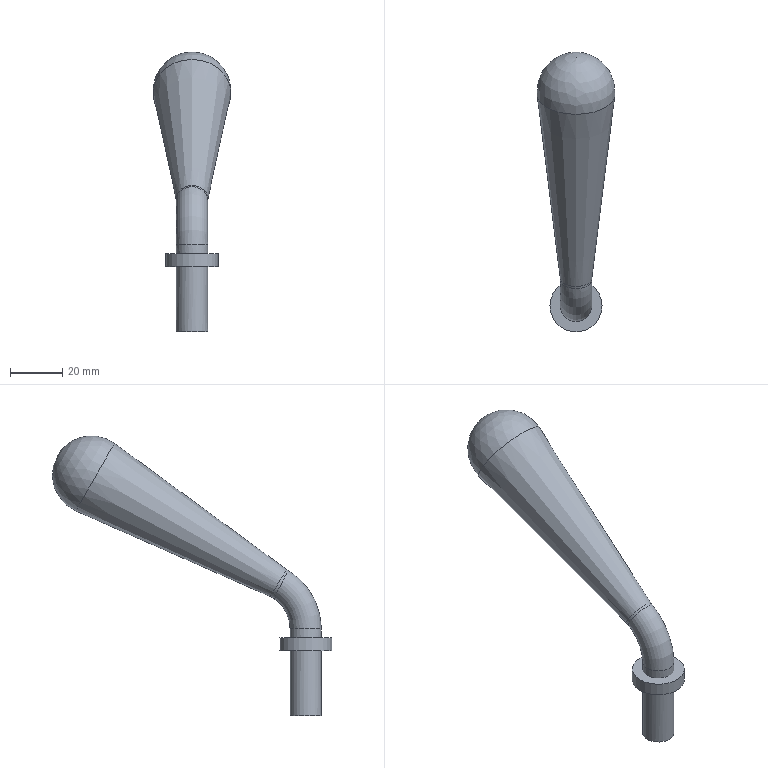Component | NX | LOCK_HANDLE | 1 solid | 10 faces | box 30 x 107.27 x 107.5 mm | volume 45177 mm3 | cylinder 3 | plane 3 | torus 1 | sphere 1 | cone 1 | spline 1 | commonest cylinder face diameters 12 x2 20 x1
STEP:
#1=CARTESIAN_POINT('',(0.,0.,0.));
#2=DIRECTION('',(0.,0.,1.));
#3=DIRECTION('',(1.,0.,0.));
#4=AXIS2_PLACEMENT_3D('',#1,#2,#3);
#5=CARTESIAN_POINT('',(36.,50.,164.5));
#6=VERTEX_POINT('',#5);
#7=CARTESIAN_POINT('',(42.,44.,164.5));
#8=VERTEX_POINT('',#7);
#9=CARTESIAN_POINT('',(36.,44.,164.5));
#10=DIRECTION('',(0.,0.,-1.));
#11=DIRECTION('',(1.,0.,0.));
#12=AXIS2_PLACEMENT_3D('',#9,#10,#11);
#13=CIRCLE('',#12,6.);
#14=CARTESIAN_POINT('',(36.,44.,167.953));
#15=DIRECTION('',(0.,0.,-1.));
#16=DIRECTION('',(-1.,0.,0.));
#17=AXIS2_PLACEMENT_3D('',#14,#15,#16);
#18=CYLINDRICAL_SURFACE('',#17,6.);
#19=CARTESIAN_POINT('',(-3.142,3.453));
#20=DIRECTION('',(1.,0.));
#21=VECTOR('',#20,1.);
#22=LINE('',#19,#21);
#23=(GEOMETRIC_REPRESENTATION_CONTEXT(2)PARAMETRIC_REPRESENTATION_CONTEXT()REPRESENTATION_CONTEXT('',''));
#24=DEFINITIONAL_REPRESENTATION('',(#22),#23);
#25=PCURVE('',#18,#24);
#26=CARTESIAN_POINT('',(36.,44.,164.5));
#27=DIRECTION('',(0.,0.,1.));
#28=DIRECTION('',(1.,0.,0.));
#29=AXIS2_PLACEMENT_3D('',#26,#27,#28);
#30=PLANE('',#29);
#31=CARTESIAN_POINT('',(6.,0.));
#32=CARTESIAN_POINT('',(6.,-10.392));
#33=CARTESIAN_POINT('',(-3.,-5.196));
#34=CARTESIAN_POINT('',(-12.,-0.));
#35=CARTESIAN_POINT('',(-3.,5.196));
#36=CARTESIAN_POINT('',(6.,10.392));
#37=CARTESIAN_POINT('',(6.,0.));
#38=(BOUNDED_CURVE()B_SPLINE_CURVE(2,(#31,#32,#33,#34,#35,#36,#37),.UNSPECIFIED.,.T.,.F.)B_SPLINE_CURVE_WITH_KNOTS((1,2,2,2,2,1),(-2.094,0.,2.094,4.189,6.283,8.378),.UNSPECIFIED.)CURVE()GEOMETRIC_REPRESENTATION_ITEM()RATIONAL_B_SPLINE_CURVE((1.,0.5,1.,0.5,1.,0.5,1.))REPRESENTATION_ITEM(''));
#39=(GEOMETRIC_REPRESENTATION_CONTEXT(2)PARAMETRIC_REPRESENTATION_CONTEXT()REPRESENTATION_CONTEXT('',''));
#40=DEFINITIONAL_REPRESENTATION('',(#38),#39);
#41=PCURVE('',#30,#40);
#42=SURFACE_CURVE('',#13,(#25,#41),.PCURVE_S1.);
#43=EDGE_CURVE('',#6,#8,#42,.T.);
#44=ORIENTED_EDGE('',*,*,#43,.F.);
#45=CARTESIAN_POINT('',(36.,50.,167.953));
#46=VERTEX_POINT('',#45);
#47=CARTESIAN_POINT('',(36.,50.,167.953));
#48=CARTESIAN_POINT('',(36.,50.,164.5));
#49=B_SPLINE_CURVE_WITH_KNOTS('',1,(#47,#48),.UNSPECIFIED.,.F.,.F.,(2,2),(0.,3.453),.PIECEWISE_BEZIER_KNOTS.);
#50=CARTESIAN_POINT('',(1.571,0.));
#51=DIRECTION('',(0.,1.));
#52=VECTOR('',#51,1.);
#53=LINE('',#50,#52);
#54=(GEOMETRIC_REPRESENTATION_CONTEXT(2)PARAMETRIC_REPRESENTATION_CONTEXT()REPRESENTATION_CONTEXT('',''));
#55=DEFINITIONAL_REPRESENTATION('',(#53),#54);
#56=PCURVE('',#18,#55);
#57=CARTESIAN_POINT('',(7.854,0.));
#58=DIRECTION('',(0.,1.));
#59=VECTOR('',#58,1.);
#60=LINE('',#57,#59);
#61=(GEOMETRIC_REPRESENTATION_CONTEXT(2)PARAMETRIC_REPRESENTATION_CONTEXT()REPRESENTATION_CONTEXT('',''));
#62=DEFINITIONAL_REPRESENTATION('',(#60),#61);
#63=PCURVE('',#18,#62);
#64=SEAM_CURVE('',#49,(#56,#63),.PCURVE_S1.);
#65=EDGE_CURVE('',#46,#6,#64,.T.);
#66=ORIENTED_EDGE('',*,*,#65,.F.);
#67=CARTESIAN_POINT('',(36.,38.,167.953));
#68=VERTEX_POINT('',#67);
#69=CARTESIAN_POINT('',(36.,44.,167.953));
#70=DIRECTION('',(0.,-0.,-1.));
#71=DIRECTION('',(0.,1.,-0.));
#72=AXIS2_PLACEMENT_3D('',#69,#70,#71);
#73=CIRCLE('',#72,6.);
#74=CARTESIAN_POINT('',(1.571,0.));
#75=DIRECTION('',(1.,0.));
#76=VECTOR('',#75,1.);
#77=LINE('',#74,#76);
#78=(GEOMETRIC_REPRESENTATION_CONTEXT(2)PARAMETRIC_REPRESENTATION_CONTEXT()REPRESENTATION_CONTEXT('',''));
#79=DEFINITIONAL_REPRESENTATION('',(#77),#78);
#80=PCURVE('',#18,#79);
#81=CARTESIAN_POINT('',(36.,64.,167.953));
#82=DIRECTION('',(-1.,0.,0.));
#83=DIRECTION('',(0.,0.,1.));
#84=AXIS2_PLACEMENT_3D('',#81,#82,#83);
#85=TOROIDAL_SURFACE('',#84,20.,6.);
#86=CARTESIAN_POINT('',(4.712,3.142));
#87=DIRECTION('',(0.,1.));
#88=VECTOR('',#87,1.);
#89=LINE('',#86,#88);
#90=(GEOMETRIC_REPRESENTATION_CONTEXT(2)PARAMETRIC_REPRESENTATION_CONTEXT()REPRESENTATION_CONTEXT('',''));
#91=DEFINITIONAL_REPRESENTATION('',(#89),#90);
#92=PCURVE('',#85,#91);
#93=SURFACE_CURVE('',#73,(#80,#92),.PCURVE_S1.);
#94=EDGE_CURVE('',#46,#68,#93,.T.);
#95=ORIENTED_EDGE('',*,*,#94,.T.);
#96=CARTESIAN_POINT('',(36.,44.,167.953));
#97=DIRECTION('',(0.,-0.,-1.));
#98=DIRECTION('',(0.,1.,-0.));
#99=AXIS2_PLACEMENT_3D('',#96,#97,#98);
#100=CIRCLE('',#99,6.);
#101=CARTESIAN_POINT('',(1.571,0.));
#102=DIRECTION('',(1.,0.));
#103=VECTOR('',#102,1.);
#104=LINE('',#101,#103);
#105=(GEOMETRIC_REPRESENTATION_CONTEXT(2)PARAMETRIC_REPRESENTATION_CONTEXT()REPRESENTATION_CONTEXT('',''));
#106=DEFINITIONAL_REPRESENTATION('',(#104),#105);
#107=PCURVE('',#18,#106);
#108=CARTESIAN_POINT('',(4.712,-3.142));
#109=DIRECTION('',(0.,1.));
#110=VECTOR('',#109,1.);
#111=LINE('',#108,#110);
#112=(GEOMETRIC_REPRESENTATION_CONTEXT(2)PARAMETRIC_REPRESENTATION_CONTEXT()REPRESENTATION_CONTEXT('',''));
#113=DEFINITIONAL_REPRESENTATION('',(#111),#112);
#114=PCURVE('',#85,#113);
#115=SURFACE_CURVE('',#100,(#107,#114),.PCURVE_S1.);
#116=EDGE_CURVE('',#68,#46,#115,.T.);
#117=ORIENTED_EDGE('',*,*,#116,.T.);
#118=ORIENTED_EDGE('',*,*,#65,.T.);
#119=CARTESIAN_POINT('',(36.,44.,164.5));
#120=DIRECTION('',(0.,0.,-1.));
#121=DIRECTION('',(1.,0.,0.));
#122=AXIS2_PLACEMENT_3D('',#119,#120,#121);
#123=CIRCLE('',#122,6.);
#124=CARTESIAN_POINT('',(3.142,3.453));
#125=DIRECTION('',(1.,0.));
#126=VECTOR('',#125,1.);
#127=LINE('',#124,#126);
#128=(GEOMETRIC_REPRESENTATION_CONTEXT(2)PARAMETRIC_REPRESENTATION_CONTEXT()REPRESENTATION_CONTEXT('',''));
#129=DEFINITIONAL_REPRESENTATION('',(#127),#128);
#130=PCURVE('',#18,#129);
#131=CARTESIAN_POINT('',(6.,0.));
#132=CARTESIAN_POINT('',(6.,-10.392));
#133=CARTESIAN_POINT('',(-3.,-5.196));
#134=CARTESIAN_POINT('',(-12.,-0.));
#135=CARTESIAN_POINT('',(-3.,5.196));
#136=CARTESIAN_POINT('',(6.,10.392));
#137=CARTESIAN_POINT('',(6.,0.));
#138=(BOUNDED_CURVE()B_SPLINE_CURVE(2,(#131,#132,#133,#134,#135,#136,#137),.UNSPECIFIED.,.T.,.F.)B_SPLINE_CURVE_WITH_KNOTS((1,2,2,2,2,1),(-2.094,0.,2.094,4.189,6.283,8.378),.UNSPECIFIED.)CURVE()GEOMETRIC_REPRESENTATION_ITEM()RATIONAL_B_SPLINE_CURVE((1.,0.5,1.,0.5,1.,0.5,1.))REPRESENTATION_ITEM(''));
#139=(GEOMETRIC_REPRESENTATION_CONTEXT(2)PARAMETRIC_REPRESENTATION_CONTEXT()REPRESENTATION_CONTEXT('',''));
#140=DEFINITIONAL_REPRESENTATION('',(#138),#139);
#141=PCURVE('',#30,#140);
#142=SURFACE_CURVE('',#123,(#130,#141),.PCURVE_S1.);
#143=EDGE_CURVE('',#8,#6,#142,.T.);
#144=ORIENTED_EDGE('',*,*,#143,.F.);
#145=EDGE_LOOP('',(#44,#66,#95,#117,#118,#144));
#146=FACE_BOUND('',#145,.T.);
#147=ADVANCED_FACE('',(#146),#18,.T.);
#148=CARTESIAN_POINT('',(36.,50.635,190.255));
#149=VERTEX_POINT('',#148);
#150=CARTESIAN_POINT('',(37.592,50.635,190.255));
#151=CARTESIAN_POINT('',(34.408,50.635,190.255));
#152=CARTESIAN_POINT('',(32.847,50.958,189.681));
#153=CARTESIAN_POINT('',(30.634,52.045,187.731));
#154=CARTESIAN_POINT('',(29.99,52.804,186.366));
#155=CARTESIAN_POINT('',(30.01,54.3,183.557));
#156=CARTESIAN_POINT('',(30.675,55.003,182.174));
#157=CARTESIAN_POINT('',(32.89,55.827,180.099));
#158=CARTESIAN_POINT('',(34.423,55.885,179.356));
#159=CARTESIAN_POINT('',(37.609,55.884,179.366));
#160=CARTESIAN_POINT('',(39.13,55.824,180.111));
#161=CARTESIAN_POINT('',(41.334,54.995,182.189));
#162=CARTESIAN_POINT('',(41.993,54.285,183.586));
#163=CARTESIAN_POINT('',(42.007,52.809,186.356));
#164=CARTESIAN_POINT('',(41.375,52.049,187.725));
#165=CARTESIAN_POINT('',(39.136,50.951,189.693));
#166=CARTESIAN_POINT('',(37.592,50.635,190.255));
#167=CARTESIAN_POINT('',(34.408,50.635,190.255));
#168=B_SPLINE_CURVE_WITH_KNOTS('',3,(#150,#151,#152,#153,#154,#155,#156,#157,#158,#159,#160,#161,#162,#163,#164,#165,#166,#167),.UNSPECIFIED.,.T.,.F.,(2,2,2,2,2,2,2,2,2,2,2),(-0.125,0.,0.125,0.25,0.375,0.5,0.625,0.75,0.875,1.,1.125),.UNSPECIFIED.);
#169=CARTESIAN_POINT('',(5.743,0.));
#170=CARTESIAN_POINT('',(5.743,0.04821));
#171=CARTESIAN_POINT('',(5.743,0.1444));
#172=CARTESIAN_POINT('',(5.743,0.2882));
#173=CARTESIAN_POINT('',(5.743,0.4318));
#174=CARTESIAN_POINT('',(5.742,0.575));
#175=CARTESIAN_POINT('',(5.742,0.7179));
#176=CARTESIAN_POINT('',(5.741,0.8607));
#177=CARTESIAN_POINT('',(5.74,1.003));
#178=CARTESIAN_POINT('',(5.738,1.146));
#179=CARTESIAN_POINT('',(5.737,1.29));
#180=CARTESIAN_POINT('',(5.735,1.433));
#181=CARTESIAN_POINT('',(5.732,1.577));
#182=CARTESIAN_POINT('',(5.729,1.721));
#183=CARTESIAN_POINT('',(5.726,1.864));
#184=CARTESIAN_POINT('',(5.722,2.007));
#185=CARTESIAN_POINT('',(5.716,2.15));
#186=CARTESIAN_POINT('',(5.71,2.291));
#187=CARTESIAN_POINT('',(5.702,2.433));
#188=CARTESIAN_POINT('',(5.693,2.574));
#189=CARTESIAN_POINT('',(5.683,2.716));
#190=CARTESIAN_POINT('',(5.673,2.858));
#191=CARTESIAN_POINT('',(5.667,3.));
#192=CARTESIAN_POINT('',(5.664,3.144));
#193=CARTESIAN_POINT('',(5.667,3.288));
#194=CARTESIAN_POINT('',(5.674,3.43));
#195=CARTESIAN_POINT('',(5.683,3.572));
#196=CARTESIAN_POINT('',(5.693,3.713));
#197=CARTESIAN_POINT('',(5.702,3.854));
#198=CARTESIAN_POINT('',(5.71,3.995));
#199=CARTESIAN_POINT('',(5.716,4.137));
#200=CARTESIAN_POINT('',(5.722,4.28));
#201=CARTESIAN_POINT('',(5.726,4.423));
#202=CARTESIAN_POINT('',(5.73,4.565));
#203=CARTESIAN_POINT('',(5.732,4.708));
#204=CARTESIAN_POINT('',(5.735,4.85));
#205=CARTESIAN_POINT('',(5.737,4.993));
#206=CARTESIAN_POINT('',(5.738,5.136));
#207=CARTESIAN_POINT('',(5.74,5.279));
#208=CARTESIAN_POINT('',(5.741,5.423));
#209=CARTESIAN_POINT('',(5.742,5.567));
#210=CARTESIAN_POINT('',(5.742,5.71));
#211=CARTESIAN_POINT('',(5.743,5.853));
#212=CARTESIAN_POINT('',(5.743,5.996));
#213=CARTESIAN_POINT('',(5.743,6.139));
#214=CARTESIAN_POINT('',(5.743,6.235));
#215=CARTESIAN_POINT('',(5.743,6.283));
#216=B_SPLINE_CURVE_WITH_KNOTS('',3,(#169,#170,#171,#172,#173,#174,#175,#176,#177,#178,#179,#180,#181,#182,#183,#184,#185,#186,#187,#188,#189,#190,#191,#192,#193,#194,#195,#196,#197,#198,#199,#200,#201,#202,#203,#204,#205,#206,#207,#208,#209,#210,#211,#212,#213,#214,#215),.UNSPECIFIED.,.F.,.F.,(4,1,1,1,1,1,1,1,1,1,1,1,1,1,1,1,1,1,1,1,1,1,1,1,1,1,1,1,1,1,1,1,1,1,1,1,1,1,1,1,1,1,1,1,4),(0.,0.02273,0.04545,0.06818,0.09091,0.1136,0.1364,0.1591,0.1818,0.2045,0.2273,0.25,0.2727,0.2955,0.3182,0.3409,0.3636,0.3864,0.4091,0.4318,0.4545,0.4773,0.5,0.5227,0.5455,0.5682,0.5909,0.6136,0.6364,0.6591,0.6818,0.7045,0.7273,0.75,0.7727,0.7955,0.8182,0.8409,0.8636,0.8864,0.9091,0.9318,0.9545,0.9773,1.),.QUASI_UNIFORM_KNOTS.);
#217=(GEOMETRIC_REPRESENTATION_CONTEXT(2)PARAMETRIC_REPRESENTATION_CONTEXT()REPRESENTATION_CONTEXT('',''));
#218=DEFINITIONAL_REPRESENTATION('',(#216),#217);
#219=PCURVE('',#85,#218);
#220=CARTESIAN_POINT('',(36.634,50.651,190.225));
#221=CARTESIAN_POINT('',(36.635,51.047,190.463));
#222=CARTESIAN_POINT('',(36.64,51.42,190.735));
#223=CARTESIAN_POINT('',(37.423,50.692,190.152));
#224=CARTESIAN_POINT('',(37.425,51.089,190.39));
#225=CARTESIAN_POINT('',(37.436,51.462,190.662));
#226=CARTESIAN_POINT('',(38.18,50.809,189.945));
#227=CARTESIAN_POINT('',(38.183,51.207,190.183));
#228=CARTESIAN_POINT('',(38.2,51.583,190.455));
#229=CARTESIAN_POINT('',(39.216,51.085,189.452));
#230=CARTESIAN_POINT('',(39.22,51.488,189.692));
#231=CARTESIAN_POINT('',(39.246,51.87,189.963));
#232=CARTESIAN_POINT('',(39.54,51.192,189.26));
#233=CARTESIAN_POINT('',(39.543,51.597,189.501));
#234=CARTESIAN_POINT('',(39.573,51.982,189.771));
#235=CARTESIAN_POINT('',(40.142,51.437,188.822));
#236=CARTESIAN_POINT('',(40.146,51.847,189.064));
#237=CARTESIAN_POINT('',(40.181,52.238,189.334));
#238=CARTESIAN_POINT('',(40.422,51.576,188.573));
#239=CARTESIAN_POINT('',(40.426,51.989,188.817));
#240=CARTESIAN_POINT('',(40.464,52.383,189.086));
#241=CARTESIAN_POINT('',(41.16,52.02,187.774));
#242=CARTESIAN_POINT('',(41.164,52.442,188.022));
#243=CARTESIAN_POINT('',(41.209,52.849,188.29));
#244=CARTESIAN_POINT('',(41.534,52.366,187.15));
#245=CARTESIAN_POINT('',(41.537,52.796,187.401));
#246=CARTESIAN_POINT('',(41.587,53.213,187.669));
#247=CARTESIAN_POINT('',(41.976,53.085,185.833));
#248=CARTESIAN_POINT('',(41.978,53.537,186.096));
#249=CARTESIAN_POINT('',(42.034,53.981,186.365));
#250=CARTESIAN_POINT('',(42.049,53.467,185.126));
#251=CARTESIAN_POINT('',(42.05,53.932,185.397));
#252=CARTESIAN_POINT('',(42.108,54.393,185.668));
#253=CARTESIAN_POINT('',(41.884,54.193,183.746));
#254=CARTESIAN_POINT('',(41.881,54.692,184.038));
#255=CARTESIAN_POINT('',(41.943,55.196,184.316));
#256=CARTESIAN_POINT('',(41.647,54.542,183.061));
#257=CARTESIAN_POINT('',(41.641,55.063,183.368));
#258=CARTESIAN_POINT('',(41.704,55.594,183.652));
#259=CARTESIAN_POINT('',(40.896,55.14,181.806));
#260=CARTESIAN_POINT('',(40.884,55.717,182.155));
#261=CARTESIAN_POINT('',(40.947,56.317,182.457));
#262=CARTESIAN_POINT('',(40.388,55.387,181.238));
#263=CARTESIAN_POINT('',(40.373,55.998,181.615));
#264=CARTESIAN_POINT('',(40.435,56.642,181.93));
#265=CARTESIAN_POINT('',(39.157,55.732,180.273));
#266=CARTESIAN_POINT('',(39.138,56.428,180.725));
#267=CARTESIAN_POINT('',(39.192,57.179,181.075));
#268=CARTESIAN_POINT('',(38.454,55.82,179.888));
#269=CARTESIAN_POINT('',(38.433,56.566,180.388));
#270=CARTESIAN_POINT('',(38.482,57.383,180.76));
#271=CARTESIAN_POINT('',(36.944,55.892,179.394));
#272=CARTESIAN_POINT('',(36.932,56.714,179.975));
#273=CARTESIAN_POINT('',(36.955,57.634,180.382));
#274=CARTESIAN_POINT('',(36.15,55.889,179.303));
#275=CARTESIAN_POINT('',(36.149,56.73,179.905));
#276=CARTESIAN_POINT('',(36.151,57.677,180.321));
#277=CARTESIAN_POINT('',(34.581,55.875,179.498));
#278=CARTESIAN_POINT('',(34.597,56.682,180.062));
#279=CARTESIAN_POINT('',(34.565,57.581,180.462));
#280=CARTESIAN_POINT('',(33.82,55.85,179.771));
#281=CARTESIAN_POINT('',(33.84,56.611,180.285));
#282=CARTESIAN_POINT('',(33.795,57.446,180.663));
#283=CARTESIAN_POINT('',(32.438,55.645,180.541));
#284=CARTESIAN_POINT('',(32.457,56.315,180.969));
#285=CARTESIAN_POINT('',(32.399,57.032,181.307));
#286=CARTESIAN_POINT('',(31.828,55.468,181.032));
#287=CARTESIAN_POINT('',(31.844,56.095,181.422));
#288=CARTESIAN_POINT('',(31.783,56.757,181.743));
#289=CARTESIAN_POINT('',(30.834,54.971,182.178));
#290=CARTESIAN_POINT('',(30.844,55.529,182.511));
#291=CARTESIAN_POINT('',(30.78,56.104,182.807));
#292=CARTESIAN_POINT('',(30.466,54.662,182.815));
#293=CARTESIAN_POINT('',(30.473,55.193,183.129));
#294=CARTESIAN_POINT('',(30.41,55.736,183.416));
#295=CARTESIAN_POINT('',(30.022,53.977,184.165));
#296=CARTESIAN_POINT('',(30.024,54.464,184.449));
#297=CARTESIAN_POINT('',(29.963,54.953,184.724));
#298=CARTESIAN_POINT('',(29.951,53.602,184.871));
#299=CARTESIAN_POINT('',(29.951,54.073,185.146));
#300=CARTESIAN_POINT('',(29.892,54.541,185.418));
#301=CARTESIAN_POINT('',(30.117,52.863,186.244));
#302=CARTESIAN_POINT('',(30.114,53.307,186.502));
#303=CARTESIAN_POINT('',(30.06,53.742,186.771));
#304=CARTESIAN_POINT('',(30.357,52.493,186.918));
#305=CARTESIAN_POINT('',(30.354,52.926,187.172));
#306=CARTESIAN_POINT('',(30.303,53.349,187.44));
#307=CARTESIAN_POINT('',(31.104,51.828,188.121));
#308=CARTESIAN_POINT('',(31.1,52.246,188.366));
#309=CARTESIAN_POINT('',(31.058,52.647,188.635));
#310=CARTESIAN_POINT('',(31.62,51.527,188.661));
#311=CARTESIAN_POINT('',(31.616,51.939,188.904));
#312=CARTESIAN_POINT('',(31.579,52.332,189.174));
#313=CARTESIAN_POINT('',(32.533,51.167,189.306));
#314=CARTESIAN_POINT('',(32.53,51.572,189.546));
#315=CARTESIAN_POINT('',(32.501,51.956,189.817));
#316=CARTESIAN_POINT('',(32.867,51.059,189.497));
#317=CARTESIAN_POINT('',(32.864,51.462,189.737));
#318=CARTESIAN_POINT('',(32.838,51.844,190.008));
#319=CARTESIAN_POINT('',(33.562,50.881,189.815));
#320=CARTESIAN_POINT('',(33.559,51.281,190.054));
#321=CARTESIAN_POINT('',(33.539,51.659,190.325));
#322=CARTESIAN_POINT('',(33.924,50.809,189.943));
#323=CARTESIAN_POINT('',(33.922,51.208,190.182));
#324=CARTESIAN_POINT('',(33.905,51.584,190.453));
#325=CARTESIAN_POINT('',(35.056,50.646,190.235));
#326=CARTESIAN_POINT('',(35.055,51.042,190.472));
#327=CARTESIAN_POINT('',(35.047,51.414,190.744));
#328=CARTESIAN_POINT('',(35.846,50.61,190.299));
#329=CARTESIAN_POINT('',(35.846,51.005,190.535));
#330=CARTESIAN_POINT('',(35.845,51.377,190.808));
#331=CARTESIAN_POINT('',(36.634,50.651,190.225));
#332=CARTESIAN_POINT('',(36.635,51.047,190.463));
#333=CARTESIAN_POINT('',(36.64,51.42,190.735));
#334=(BOUNDED_SURFACE()B_SPLINE_SURFACE(3,2,((#220,#221,#222),(#223,#224,#225),(#226,#227,#228),(#229,#230,#231),(#232,#233,#234),(#235,#236,#237),(#238,#239,#240),(#241,#242,#243),(#244,#245,#246),(#247,#248,#249),(#250,#251,#252),(#253,#254,#255),(#256,#257,#258),(#259,#260,#261),(#262,#263,#264),(#265,#266,#267),(#268,#269,#270),(#271,#272,#273),(#274,#275,#276),(#277,#278,#279),(#280,#281,#282),(#283,#284,#285),(#286,#287,#288),(#289,#290,#291),(#292,#293,#294),(#295,#296,#297),(#298,#299,#300),(#301,#302,#303),(#304,#305,#306),(#307,#308,#309),(#310,#311,#312),(#313,#314,#315),(#316,#317,#318),(#319,#320,#321),(#322,#323,#324),(#325,#326,#327),(#328,#329,#330),(#331,#332,#333)),.UNSPECIFIED.,.T.,.F.,.F.)B_SPLINE_SURFACE_WITH_KNOTS((1,3,2,2,2,2,2,2,2,2,2,2,2,2,2,2,2,2,2,3,1),(3,3),(-0.0625,0.,0.0625,0.09375,0.125,0.1875,0.25,0.3125,0.375,0.4375,0.5,0.5625,0.625,0.6875,0.75,0.8125,0.875,0.9062,0.9375,1.,1.062),(0.,1.),.UNSPECIFIED.)GEOMETRIC_REPRESENTATION_ITEM()RATIONAL_B_SPLINE_SURFACE(((1.,0.9989,1.),(1.,0.9989,1.),(1.,0.9989,1.),(1.,0.9989,1.),(1.,0.9989,1.),(1.,0.9989,1.),(1.,0.9989,1.),(1.,0.9988,1.),(1.,0.9988,1.),(1.,0.9986,1.),(1.,0.9986,1.),(1.,0.9983,1.),(1.,0.9982,1.),(1.,0.9977,1.),(1.,0.9974,1.),(1.,0.9966,1.),(1.,0.996,1.),(1.,0.995,1.),(1.,0.9947,1.),(1.,0.9952,1.),(1.,0.9958,1.),(1.,0.9969,1.),(1.,0.9973,1.),(1.,0.9979,1.),(1.,0.9981,1.),(1.,0.9984,1.),(1.,0.9985,1.),(1.,0.9987,1.),(1.,0.9987,1.),(1.,0.9988,1.),(1.,0.9989,1.),(1.,0.9989,1.),(1.,0.9989,1.),(1.,0.9989,1.),(1.,0.9989,1.),(1.,0.9989,1.),(1.,0.9989,1.),(1.,0.9989,1.)))REPRESENTATION_ITEM('')SURFACE());
#335=CARTESIAN_POINT('',(1.983,-0.00001083));
#336=CARTESIAN_POINT('',(1.976,-0.00001702));
#337=CARTESIAN_POINT('',(1.96,-0.00000151));
#338=CARTESIAN_POINT('',(1.937,0.00005651));
#339=CARTESIAN_POINT('',(1.914,0.0000587));
#340=CARTESIAN_POINT('',(1.892,0.00006053));
#341=CARTESIAN_POINT('',(1.869,0.00000074));
#342=CARTESIAN_POINT('',(1.846,-0.00000105));
#343=CARTESIAN_POINT('',(1.823,0.0002518));
#344=CARTESIAN_POINT('',(1.801,0.0004468));
#345=CARTESIAN_POINT('',(1.778,0.0004159));
#346=CARTESIAN_POINT('',(1.755,0.0001863));
#347=CARTESIAN_POINT('',(1.732,-0.00009378));
#348=CARTESIAN_POINT('',(1.709,0.00002888));
#349=CARTESIAN_POINT('',(1.686,0.0001407));
#350=CARTESIAN_POINT('',(1.664,-0.00002189));
#351=CARTESIAN_POINT('',(1.641,-0.00005329));
#352=CARTESIAN_POINT('',(1.618,-0.0000936));
#353=CARTESIAN_POINT('',(1.596,0.0006567));
#354=CARTESIAN_POINT('',(1.573,-0.006669));
#355=CARTESIAN_POINT('',(1.551,-0.008641));
#356=CARTESIAN_POINT('',(1.528,-0.005146));
#357=CARTESIAN_POINT('',(1.506,-0.0005596));
#358=CARTESIAN_POINT('',(1.483,-0.0007037));
#359=CARTESIAN_POINT('',(1.46,-0.002364));
#360=CARTESIAN_POINT('',(1.437,-0.005809));
#361=CARTESIAN_POINT('',(1.415,-0.008217));
#362=CARTESIAN_POINT('',(1.392,-0.006143));
#363=CARTESIAN_POINT('',(1.37,-0.0002228));
#364=CARTESIAN_POINT('',(1.347,0.0002452));
#365=CARTESIAN_POINT('',(1.325,-0.00008067));
#366=CARTESIAN_POINT('',(1.302,-0.00002753));
#367=CARTESIAN_POINT('',(1.279,-0.00001283));
#368=CARTESIAN_POINT('',(1.257,0.00005802));
#369=CARTESIAN_POINT('',(1.234,-0.0000647));
#370=CARTESIAN_POINT('',(1.211,0.0001232));
#371=CARTESIAN_POINT('',(1.189,0.0003692));
#372=CARTESIAN_POINT('',(1.166,0.0003632));
#373=CARTESIAN_POINT('',(1.143,0.0002114));
#374=CARTESIAN_POINT('',(1.12,-0.00000281));
#375=CARTESIAN_POINT('',(1.097,0.00000372));
#376=CARTESIAN_POINT('',(1.074,0.0001132));
#377=CARTESIAN_POINT('',(1.052,0.0001687));
#378=CARTESIAN_POINT('',(1.029,0.0001131));
#379=CARTESIAN_POINT('',(1.006,0.00005113));
#380=CARTESIAN_POINT('',(0.9908,0.00000684));
#381=CARTESIAN_POINT('',(0.9832,-0.00001083));
#382=B_SPLINE_CURVE_WITH_KNOTS('',3,(#335,#336,#337,#338,#339,#340,#341,#342,#343,#344,#345,#346,#347,#348,#349,#350,#351,#352,#353,#354,#355,#356,#357,#358,#359,#360,#361,#362,#363,#364,#365,#366,#367,#368,#369,#370,#371,#372,#373,#374,#375,#376,#377,#378,#379,#380,#381),.UNSPECIFIED.,.F.,.F.,(4,1,1,1,1,1,1,1,1,1,1,1,1,1,1,1,1,1,1,1,1,1,1,1,1,1,1,1,1,1,1,1,1,1,1,1,1,1,1,1,1,1,1,1,4),(0.,0.02273,0.04545,0.06818,0.09091,0.1136,0.1364,0.1591,0.1818,0.2045,0.2273,0.25,0.2727,0.2955,0.3182,0.3409,0.3636,0.3864,0.4091,0.4318,0.4545,0.4773,0.5,0.5227,0.5455,0.5682,0.5909,0.6136,0.6364,0.6591,0.6818,0.7045,0.7273,0.75,0.7727,0.7955,0.8182,0.8409,0.8636,0.8864,0.9091,0.9318,0.9545,0.9773,1.),.QUASI_UNIFORM_KNOTS.);
#383=(GEOMETRIC_REPRESENTATION_CONTEXT(2)PARAMETRIC_REPRESENTATION_CONTEXT()REPRESENTATION_CONTEXT('',''));
#384=DEFINITIONAL_REPRESENTATION('',(#382),#383);
#385=PCURVE('',#334,#384);
#386=SURFACE_CURVE('',#168,(#219,#385),.PCURVE_S1.);
#387=EDGE_CURVE('',#149,#149,#386,.T.);
#388=ORIENTED_EDGE('',*,*,#387,.T.);
#389=CARTESIAN_POINT('',(36.,38.,167.953));
#390=CARTESIAN_POINT('',(36.,38.,172.46));
#391=CARTESIAN_POINT('',(36.,38.934,176.918));
#392=CARTESIAN_POINT('',(36.,40.77,181.113));
#393=CARTESIAN_POINT('',(36.,43.425,184.845));
#394=CARTESIAN_POINT('',(36.,46.769,187.938));
#395=CARTESIAN_POINT('',(36.,50.635,190.255));
#396=(BOUNDED_CURVE()B_SPLINE_CURVE(6,(#389,#390,#391,#392,#393,#394,#395),.UNSPECIFIED.,.F.,.F.)B_SPLINE_CURVE_WITH_KNOTS((7,7),(4.712,5.743),.PIECEWISE_BEZIER_KNOTS.)CURVE()GEOMETRIC_REPRESENTATION_ITEM()RATIONAL_B_SPLINE_CURVE((1.013,1.004,0.9991,0.9974,0.9991,1.004,1.013))REPRESENTATION_ITEM(''));
#397=CARTESIAN_POINT('',(0.,6.283));
#398=DIRECTION('',(1.,0.));
#399=VECTOR('',#398,1.);
#400=LINE('',#397,#399);
#401=(GEOMETRIC_REPRESENTATION_CONTEXT(2)PARAMETRIC_REPRESENTATION_CONTEXT()REPRESENTATION_CONTEXT('',''));
#402=DEFINITIONAL_REPRESENTATION('',(#400),#401);
#403=PCURVE('',#85,#402);
#404=CARTESIAN_POINT('',(0.,0.));
#405=DIRECTION('',(1.,0.));
#406=VECTOR('',#405,1.);
#407=LINE('',#404,#406);
#408=(GEOMETRIC_REPRESENTATION_CONTEXT(2)PARAMETRIC_REPRESENTATION_CONTEXT()REPRESENTATION_CONTEXT('',''));
#409=DEFINITIONAL_REPRESENTATION('',(#407),#408);
#410=PCURVE('',#85,#409);
#411=SEAM_CURVE('',#396,(#403,#410),.PCURVE_S1.);
#412=EDGE_CURVE('',#68,#149,#411,.T.);
#413=ORIENTED_EDGE('',*,*,#412,.F.);
#414=ORIENTED_EDGE('',*,*,#94,.F.);
#415=ORIENTED_EDGE('',*,*,#116,.F.);
#416=ORIENTED_EDGE('',*,*,#412,.T.);
#417=EDGE_LOOP('',(#388,#413,#414,#415,#416));
#418=FACE_BOUND('',#417,.T.);
#419=ADVANCED_FACE('',(#418),#85,.T.);
#420=CARTESIAN_POINT('',(36.,117.41,239.102));
#421=VERTEX_POINT('',#420);
#422=CARTESIAN_POINT('',(36.,124.866,226.188));
#423=DIRECTION('',(0.,0.866,0.5));
#424=DIRECTION('',(0.,-0.5,0.866));
#425=AXIS2_PLACEMENT_3D('',#422,#423,#424);
#426=CIRCLE('',#425,14.912);
#427=CARTESIAN_POINT('',(36.,126.272,227.));
#428=DIRECTION('',(0.,0.866,0.5));
#429=DIRECTION('',(0.,-0.5,0.866));
#430=AXIS2_PLACEMENT_3D('',#427,#428,#429);
#431=SPHERICAL_SURFACE('',#430,15.);
#432=CARTESIAN_POINT('',(0.,-0.1085));
#433=DIRECTION('',(1.,0.));
#434=VECTOR('',#433,1.);
#435=LINE('',#432,#434);
#436=(GEOMETRIC_REPRESENTATION_CONTEXT(2)PARAMETRIC_REPRESENTATION_CONTEXT()REPRESENTATION_CONTEXT('',''));
#437=DEFINITIONAL_REPRESENTATION('',(#435),#436);
#438=PCURVE('',#431,#437);
#439=CARTESIAN_POINT('',(36.,54.,185.274));
#440=DIRECTION('',(0.,0.866,0.5));
#441=DIRECTION('',(0.,-0.5,0.866));
#442=AXIS2_PLACEMENT_3D('',#439,#440,#441);
#443=CONICAL_SURFACE('',#442,6.,0.1085);
#444=CARTESIAN_POINT('',(0.,81.829));
#445=DIRECTION('',(1.,0.));
#446=VECTOR('',#445,1.);
#447=LINE('',#444,#446);
#448=(GEOMETRIC_REPRESENTATION_CONTEXT(2)PARAMETRIC_REPRESENTATION_CONTEXT()REPRESENTATION_CONTEXT('',''));
#449=DEFINITIONAL_REPRESENTATION('',(#447),#448);
#450=PCURVE('',#443,#449);
#451=SURFACE_CURVE('',#426,(#438,#450),.PCURVE_S1.);
#452=EDGE_CURVE('',#421,#421,#451,.T.);
#453=ORIENTED_EDGE('',*,*,#452,.T.);
#454=CARTESIAN_POINT('',(36.,139.263,234.5));
#455=VERTEX_POINT('',#454);
#456=CARTESIAN_POINT('',(36.,117.41,239.102));
#457=CARTESIAN_POINT('',(36.,120.313,241.228));
#458=CARTESIAN_POINT('',(36.,123.812,242.542));
#459=CARTESIAN_POINT('',(36.,127.632,242.843));
#460=CARTESIAN_POINT('',(36.,131.418,242.046));
#461=CARTESIAN_POINT('',(36.,134.792,240.229));
#462=CARTESIAN_POINT('',(36.,137.464,237.616));
#463=CARTESIAN_POINT('',(36.,139.263,234.5));
#464=B_SPLINE_CURVE_WITH_KNOTS('',7,(#456,#457,#458,#459,#460,#461,#462,#463),.UNSPECIFIED.,.F.,.F.,(8,8),(-0.1085,1.571),.PIECEWISE_BEZIER_KNOTS.);
#465=CARTESIAN_POINT('',(6.283,0.));
#466=DIRECTION('',(0.,1.));
#467=VECTOR('',#466,1.);
#468=LINE('',#465,#467);
#469=(GEOMETRIC_REPRESENTATION_CONTEXT(2)PARAMETRIC_REPRESENTATION_CONTEXT()REPRESENTATION_CONTEXT('',''));
#470=DEFINITIONAL_REPRESENTATION('',(#468),#469);
#471=PCURVE('',#431,#470);
#472=CARTESIAN_POINT('',(0.,0.));
#473=DIRECTION('',(0.,1.));
#474=VECTOR('',#473,1.);
#475=LINE('',#472,#474);
#476=(GEOMETRIC_REPRESENTATION_CONTEXT(2)PARAMETRIC_REPRESENTATION_CONTEXT()REPRESENTATION_CONTEXT('',''));
#477=DEFINITIONAL_REPRESENTATION('',(#475),#476);
#478=PCURVE('',#431,#477);
#479=SEAM_CURVE('',#464,(#471,#478),.PCURVE_S1.);
#480=EDGE_CURVE('',#421,#455,#479,.T.);
#481=ORIENTED_EDGE('',*,*,#480,.T.);
#482=ORIENTED_EDGE('',*,*,#480,.F.);
#483=EDGE_LOOP('',(#453,#481,#482));
#484=FACE_BOUND('',#483,.T.);
#485=ADVANCED_FACE('',(#484),#431,.T.);
#486=CARTESIAN_POINT('',(36.,51.402,190.764));
#487=VERTEX_POINT('',#486);
#488=CARTESIAN_POINT('',(34.399,51.402,190.764));
#489=CARTESIAN_POINT('',(37.601,51.402,190.764));
#490=CARTESIAN_POINT('',(39.158,51.728,190.206));
#491=CARTESIAN_POINT('',(41.418,52.872,188.251));
#492=CARTESIAN_POINT('',(42.06,53.668,186.893));
#493=CARTESIAN_POINT('',(42.058,55.279,184.173));
#494=CARTESIAN_POINT('',(41.402,56.093,182.816));
#495=CARTESIAN_POINT('',(39.17,57.275,180.913));
#496=CARTESIAN_POINT('',(37.606,57.648,180.364));
#497=CARTESIAN_POINT('',(34.403,57.649,180.362));
#498=CARTESIAN_POINT('',(32.835,57.277,180.91));
#499=CARTESIAN_POINT('',(30.6,56.095,182.813));
#500=CARTESIAN_POINT('',(29.943,55.289,184.157));
#501=CARTESIAN_POINT('',(29.94,53.659,186.909));
#502=CARTESIAN_POINT('',(30.595,52.865,188.262));
#503=CARTESIAN_POINT('',(32.828,51.735,190.194));
#504=CARTESIAN_POINT('',(34.399,51.402,190.764));
#505=CARTESIAN_POINT('',(37.601,51.402,190.764));
#506=B_SPLINE_CURVE_WITH_KNOTS('',3,(#488,#489,#490,#491,#492,#493,#494,#495,#496,#497,#498,#499,#500,#501,#502,#503,#504,#505),.UNSPECIFIED.,.T.,.F.,(2,2,2,2,2,2,2,2,2,2,2),(-0.125,0.,0.125,0.25,0.375,0.5,0.625,0.75,0.875,1.,1.125),.UNSPECIFIED.);
#507=CARTESIAN_POINT('',(0.,0.4958));
#508=CARTESIAN_POINT('',(0.04808,0.4958));
#509=CARTESIAN_POINT('',(0.1438,0.4959));
#510=CARTESIAN_POINT('',(0.2867,0.4966));
#511=CARTESIAN_POINT('',(0.4292,0.4981));
#512=CARTESIAN_POINT('',(0.5719,0.5003));
#513=CARTESIAN_POINT('',(0.7149,0.5034));
#514=CARTESIAN_POINT('',(0.8591,0.507));
#515=CARTESIAN_POINT('',(1.002,0.511));
#516=CARTESIAN_POINT('',(1.145,0.5162));
#517=CARTESIAN_POINT('',(1.288,0.5226));
#518=CARTESIAN_POINT('',(1.431,0.5305));
#519=CARTESIAN_POINT('',(1.573,0.5397));
#520=CARTESIAN_POINT('',(1.715,0.5498));
#521=CARTESIAN_POINT('',(1.858,0.5617));
#522=CARTESIAN_POINT('',(2.001,0.5757));
#523=CARTESIAN_POINT('',(2.144,0.5919));
#524=CARTESIAN_POINT('',(2.286,0.6101));
#525=CARTESIAN_POINT('',(2.428,0.6297));
#526=CARTESIAN_POINT('',(2.57,0.6506));
#527=CARTESIAN_POINT('',(2.712,0.6708));
#528=CARTESIAN_POINT('',(2.855,0.6884));
#529=CARTESIAN_POINT('',(2.997,0.701));
#530=CARTESIAN_POINT('',(3.141,0.7061));
#531=CARTESIAN_POINT('',(3.284,0.701));
#532=CARTESIAN_POINT('',(3.427,0.6885));
#533=CARTESIAN_POINT('',(3.57,0.6709));
#534=CARTESIAN_POINT('',(3.712,0.6507));
#535=CARTESIAN_POINT('',(3.854,0.6298));
#536=CARTESIAN_POINT('',(3.996,0.6102));
#537=CARTESIAN_POINT('',(4.138,0.5922));
#538=CARTESIAN_POINT('',(4.281,0.5761));
#539=CARTESIAN_POINT('',(4.424,0.5621));
#540=CARTESIAN_POINT('',(4.567,0.55));
#541=CARTESIAN_POINT('',(4.71,0.5397));
#542=CARTESIAN_POINT('',(4.854,0.5304));
#543=CARTESIAN_POINT('',(4.997,0.5225));
#544=CARTESIAN_POINT('',(5.14,0.516));
#545=CARTESIAN_POINT('',(5.283,0.5109));
#546=CARTESIAN_POINT('',(5.425,0.507));
#547=CARTESIAN_POINT('',(5.567,0.5034));
#548=CARTESIAN_POINT('',(5.71,0.5002));
#549=CARTESIAN_POINT('',(5.853,0.4978));
#550=CARTESIAN_POINT('',(5.996,0.4964));
#551=CARTESIAN_POINT('',(6.139,0.4958));
#552=CARTESIAN_POINT('',(6.235,0.4958));
#553=CARTESIAN_POINT('',(6.283,0.4958));
#554=B_SPLINE_CURVE_WITH_KNOTS('',3,(#507,#508,#509,#510,#511,#512,#513,#514,#515,#516,#517,#518,#519,#520,#521,#522,#523,#524,#525,#526,#527,#528,#529,#530,#531,#532,#533,#534,#535,#536,#537,#538,#539,#540,#541,#542,#543,#544,#545,#546,#547,#548,#549,#550,#551,#552,#553),.UNSPECIFIED.,.F.,.F.,(4,1,1,1,1,1,1,1,1,1,1,1,1,1,1,1,1,1,1,1,1,1,1,1,1,1,1,1,1,1,1,1,1,1,1,1,1,1,1,1,1,1,1,1,4),(0.,0.02273,0.04545,0.06818,0.09091,0.1136,0.1364,0.1591,0.1818,0.2045,0.2273,0.25,0.2727,0.2955,0.3182,0.3409,0.3636,0.3864,0.4091,0.4318,0.4545,0.4773,0.5,0.5227,0.5455,0.5682,0.5909,0.6136,0.6364,0.6591,0.6818,0.7045,0.7273,0.75,0.7727,0.7955,0.8182,0.8409,0.8636,0.8864,0.9091,0.9318,0.9545,0.9773,1.),.QUASI_UNIFORM_KNOTS.);
#555=(GEOMETRIC_REPRESENTATION_CONTEXT(2)PARAMETRIC_REPRESENTATION_CONTEXT()REPRESENTATION_CONTEXT('',''));
#556=DEFINITIONAL_REPRESENTATION('',(#554),#555);
#557=PCURVE('',#443,#556);
#558=CARTESIAN_POINT('',(0.9832,1.));
#559=DIRECTION('',(1.,0.));
#560=VECTOR('',#559,1.);
#561=LINE('',#558,#560);
#562=(GEOMETRIC_REPRESENTATION_CONTEXT(2)PARAMETRIC_REPRESENTATION_CONTEXT()REPRESENTATION_CONTEXT('',''));
#563=DEFINITIONAL_REPRESENTATION('',(#561),#562);
#564=PCURVE('',#334,#563);
#565=SURFACE_CURVE('',#506,(#557,#564),.PCURVE_S1.);
#566=EDGE_CURVE('',#487,#487,#565,.T.);
#567=ORIENTED_EDGE('',*,*,#566,.T.);
#568=CARTESIAN_POINT('',(36.,51.402,190.764));
#569=CARTESIAN_POINT('',(36.,117.41,239.102));
#570=B_SPLINE_CURVE_WITH_KNOTS('',1,(#568,#569),.UNSPECIFIED.,.F.,.F.,(2,2),(0.4988,82.313),.PIECEWISE_BEZIER_KNOTS.);
#571=CARTESIAN_POINT('',(6.283,0.));
#572=DIRECTION('',(0.,1.));
#573=VECTOR('',#572,1.);
#574=LINE('',#571,#573);
#575=(GEOMETRIC_REPRESENTATION_CONTEXT(2)PARAMETRIC_REPRESENTATION_CONTEXT()REPRESENTATION_CONTEXT('',''));
#576=DEFINITIONAL_REPRESENTATION('',(#574),#575);
#577=PCURVE('',#443,#576);
#578=CARTESIAN_POINT('',(0.,0.));
#579=DIRECTION('',(0.,1.));
#580=VECTOR('',#579,1.);
#581=LINE('',#578,#580);
#582=(GEOMETRIC_REPRESENTATION_CONTEXT(2)PARAMETRIC_REPRESENTATION_CONTEXT()REPRESENTATION_CONTEXT('',''));
#583=DEFINITIONAL_REPRESENTATION('',(#581),#582);
#584=PCURVE('',#443,#583);
#585=SEAM_CURVE('',#570,(#577,#584),.PCURVE_S1.);
#586=EDGE_CURVE('',#487,#421,#585,.T.);
#587=ORIENTED_EDGE('',*,*,#586,.T.);
#588=ORIENTED_EDGE('',*,*,#452,.F.);
#589=ORIENTED_EDGE('',*,*,#586,.F.);
#590=EDGE_LOOP('',(#567,#587,#588,#589));
#591=FACE_BOUND('',#590,.T.);
#592=ADVANCED_FACE('',(#591),#443,.T.);
#593=CARTESIAN_POINT('',(46.,44.,164.5));
#594=VERTEX_POINT('',#593);
#595=CARTESIAN_POINT('',(36.,44.,164.5));
#596=DIRECTION('',(0.,0.,1.));
#597=DIRECTION('',(1.,0.,0.));
#598=AXIS2_PLACEMENT_3D('',#595,#596,#597);
#599=CIRCLE('',#598,10.);
#600=CARTESIAN_POINT('',(36.,44.,164.5));
#601=DIRECTION('',(0.,0.,-1.));
#602=DIRECTION('',(-1.,0.,0.));
#603=AXIS2_PLACEMENT_3D('',#600,#601,#602);
#604=CYLINDRICAL_SURFACE('',#603,10.);
#605=CARTESIAN_POINT('',(9.425,0.));
#606=DIRECTION('',(-1.,0.));
#607=VECTOR('',#606,1.);
#608=LINE('',#605,#607);
#609=(GEOMETRIC_REPRESENTATION_CONTEXT(2)PARAMETRIC_REPRESENTATION_CONTEXT()REPRESENTATION_CONTEXT('',''));
#610=DEFINITIONAL_REPRESENTATION('',(#608),#609);
#611=PCURVE('',#604,#610);
#612=CARTESIAN_POINT('',(0.,0.));
#613=DIRECTION('',(1.,0.));
#614=AXIS2_PLACEMENT_2D('',#612,#613);
#615=CIRCLE('',#614,10.);
#616=(GEOMETRIC_REPRESENTATION_CONTEXT(2)PARAMETRIC_REPRESENTATION_CONTEXT()REPRESENTATION_CONTEXT('',''));
#617=DEFINITIONAL_REPRESENTATION('',(#615),#616);
#618=PCURVE('',#30,#617);
#619=SURFACE_CURVE('',#599,(#611,#618),.PCURVE_S1.);
#620=EDGE_CURVE('',#594,#594,#619,.T.);
#621=ORIENTED_EDGE('',*,*,#620,.F.);
#622=CARTESIAN_POINT('',(46.,44.,159.5));
#623=VERTEX_POINT('',#622);
#624=CARTESIAN_POINT('',(46.,44.,164.5));
#625=CARTESIAN_POINT('',(46.,44.,159.5));
#626=B_SPLINE_CURVE_WITH_KNOTS('',1,(#624,#625),.UNSPECIFIED.,.F.,.F.,(2,2),(0.,5.),.PIECEWISE_BEZIER_KNOTS.);
#627=CARTESIAN_POINT('',(9.425,0.));
#628=DIRECTION('',(0.,1.));
#629=VECTOR('',#628,1.);
#630=LINE('',#627,#629);
#631=(GEOMETRIC_REPRESENTATION_CONTEXT(2)PARAMETRIC_REPRESENTATION_CONTEXT()REPRESENTATION_CONTEXT('',''));
#632=DEFINITIONAL_REPRESENTATION('',(#630),#631);
#633=PCURVE('',#604,#632);
#634=CARTESIAN_POINT('',(3.142,0.));
#635=DIRECTION('',(0.,1.));
#636=VECTOR('',#635,1.);
#637=LINE('',#634,#636);
#638=(GEOMETRIC_REPRESENTATION_CONTEXT(2)PARAMETRIC_REPRESENTATION_CONTEXT()REPRESENTATION_CONTEXT('',''));
#639=DEFINITIONAL_REPRESENTATION('',(#637),#638);
#640=PCURVE('',#604,#639);
#641=SEAM_CURVE('',#626,(#633,#640),.PCURVE_S1.);
#642=EDGE_CURVE('',#594,#623,#641,.T.);
#643=ORIENTED_EDGE('',*,*,#642,.T.);
#644=CARTESIAN_POINT('',(36.,44.,159.5));
#645=DIRECTION('',(0.,0.,1.));
#646=DIRECTION('',(1.,0.,0.));
#647=AXIS2_PLACEMENT_3D('',#644,#645,#646);
#648=CIRCLE('',#647,10.);
#649=CARTESIAN_POINT('',(9.425,5.));
#650=DIRECTION('',(-1.,0.));
#651=VECTOR('',#650,1.);
#652=LINE('',#649,#651);
#653=(GEOMETRIC_REPRESENTATION_CONTEXT(2)PARAMETRIC_REPRESENTATION_CONTEXT()REPRESENTATION_CONTEXT('',''));
#654=DEFINITIONAL_REPRESENTATION('',(#652),#653);
#655=PCURVE('',#604,#654);
#656=CARTESIAN_POINT('',(36.,44.,159.5));
#657=DIRECTION('',(0.,0.,1.));
#658=DIRECTION('',(1.,0.,0.));
#659=AXIS2_PLACEMENT_3D('',#656,#657,#658);
#660=PLANE('',#659);
#661=CARTESIAN_POINT('',(0.,0.));
#662=DIRECTION('',(1.,0.));
#663=AXIS2_PLACEMENT_2D('',#661,#662);
#664=CIRCLE('',#663,10.);
#665=(GEOMETRIC_REPRESENTATION_CONTEXT(2)PARAMETRIC_REPRESENTATION_CONTEXT()REPRESENTATION_CONTEXT('',''));
#666=DEFINITIONAL_REPRESENTATION('',(#664),#665);
#667=PCURVE('',#660,#666);
#668=SURFACE_CURVE('',#648,(#655,#667),.PCURVE_S1.);
#669=EDGE_CURVE('',#623,#623,#668,.T.);
#670=ORIENTED_EDGE('',*,*,#669,.T.);
#671=ORIENTED_EDGE('',*,*,#642,.F.);
#672=EDGE_LOOP('',(#621,#643,#670,#671));
#673=FACE_BOUND('',#672,.T.);
#674=ADVANCED_FACE('',(#673),#604,.T.);
#675=ORIENTED_EDGE('',*,*,#143,.T.);
#676=ORIENTED_EDGE('',*,*,#43,.T.);
#677=EDGE_LOOP('',(#675,#676));
#678=FACE_BOUND('',#677,.T.);
#679=ORIENTED_EDGE('',*,*,#620,.T.);
#680=EDGE_LOOP('',(#679));
#681=FACE_BOUND('',#680,.T.);
#682=ADVANCED_FACE('',(#678,#681),#30,.T.);
#683=CARTESIAN_POINT('',(42.,44.,159.5));
#684=VERTEX_POINT('',#683);
#685=CARTESIAN_POINT('',(36.,50.,159.5));
#686=VERTEX_POINT('',#685);
#687=CARTESIAN_POINT('',(36.,44.,159.5));
#688=DIRECTION('',(0.,0.,-1.));
#689=DIRECTION('',(1.,0.,0.));
#690=AXIS2_PLACEMENT_3D('',#687,#688,#689);
#691=CIRCLE('',#690,6.);
#692=CARTESIAN_POINT('',(6.,0.));
#693=CARTESIAN_POINT('',(6.,-10.392));
#694=CARTESIAN_POINT('',(-3.,-5.196));
#695=CARTESIAN_POINT('',(-12.,-0.));
#696=CARTESIAN_POINT('',(-3.,5.196));
#697=CARTESIAN_POINT('',(6.,10.392));
#698=CARTESIAN_POINT('',(6.,0.));
#699=(BOUNDED_CURVE()B_SPLINE_CURVE(2,(#692,#693,#694,#695,#696,#697,#698),.UNSPECIFIED.,.T.,.F.)B_SPLINE_CURVE_WITH_KNOTS((1,2,2,2,2,1),(-2.094,0.,2.094,4.189,6.283,8.378),.UNSPECIFIED.)CURVE()GEOMETRIC_REPRESENTATION_ITEM()RATIONAL_B_SPLINE_CURVE((1.,0.5,1.,0.5,1.,0.5,1.))REPRESENTATION_ITEM(''));
#700=(GEOMETRIC_REPRESENTATION_CONTEXT(2)PARAMETRIC_REPRESENTATION_CONTEXT()REPRESENTATION_CONTEXT('',''));
#701=DEFINITIONAL_REPRESENTATION('',(#699),#700);
#702=PCURVE('',#660,#701);
#703=CARTESIAN_POINT('',(36.,44.,167.953));
#704=DIRECTION('',(0.,0.,-1.));
#705=DIRECTION('',(-1.,0.,0.));
#706=AXIS2_PLACEMENT_3D('',#703,#704,#705);
#707=CYLINDRICAL_SURFACE('',#706,6.);
#708=CARTESIAN_POINT('',(3.142,8.453));
#709=DIRECTION('',(1.,0.));
#710=VECTOR('',#709,1.);
#711=LINE('',#708,#710);
#712=(GEOMETRIC_REPRESENTATION_CONTEXT(2)PARAMETRIC_REPRESENTATION_CONTEXT()REPRESENTATION_CONTEXT('',''));
#713=DEFINITIONAL_REPRESENTATION('',(#711),#712);
#714=PCURVE('',#707,#713);
#715=SURFACE_CURVE('',#691,(#702,#714),.PCURVE_S1.);
#716=EDGE_CURVE('',#684,#686,#715,.T.);
#717=ORIENTED_EDGE('',*,*,#716,.F.);
#718=CARTESIAN_POINT('',(36.,44.,159.5));
#719=DIRECTION('',(0.,0.,-1.));
#720=DIRECTION('',(1.,0.,0.));
#721=AXIS2_PLACEMENT_3D('',#718,#719,#720);
#722=CIRCLE('',#721,6.);
#723=CARTESIAN_POINT('',(6.,0.));
#724=CARTESIAN_POINT('',(6.,-10.392));
#725=CARTESIAN_POINT('',(-3.,-5.196));
#726=CARTESIAN_POINT('',(-12.,-0.));
#727=CARTESIAN_POINT('',(-3.,5.196));
#728=CARTESIAN_POINT('',(6.,10.392));
#729=CARTESIAN_POINT('',(6.,0.));
#730=(BOUNDED_CURVE()B_SPLINE_CURVE(2,(#723,#724,#725,#726,#727,#728,#729),.UNSPECIFIED.,.T.,.F.)B_SPLINE_CURVE_WITH_KNOTS((1,2,2,2,2,1),(-2.094,0.,2.094,4.189,6.283,8.378),.UNSPECIFIED.)CURVE()GEOMETRIC_REPRESENTATION_ITEM()RATIONAL_B_SPLINE_CURVE((1.,0.5,1.,0.5,1.,0.5,1.))REPRESENTATION_ITEM(''));
#731=(GEOMETRIC_REPRESENTATION_CONTEXT(2)PARAMETRIC_REPRESENTATION_CONTEXT()REPRESENTATION_CONTEXT('',''));
#732=DEFINITIONAL_REPRESENTATION('',(#730),#731);
#733=PCURVE('',#660,#732);
#734=CARTESIAN_POINT('',(-3.142,8.453));
#735=DIRECTION('',(1.,0.));
#736=VECTOR('',#735,1.);
#737=LINE('',#734,#736);
#738=(GEOMETRIC_REPRESENTATION_CONTEXT(2)PARAMETRIC_REPRESENTATION_CONTEXT()REPRESENTATION_CONTEXT('',''));
#739=DEFINITIONAL_REPRESENTATION('',(#737),#738);
#740=PCURVE('',#707,#739);
#741=SURFACE_CURVE('',#722,(#733,#740),.PCURVE_S1.);
#742=EDGE_CURVE('',#686,#684,#741,.T.);
#743=ORIENTED_EDGE('',*,*,#742,.F.);
#744=EDGE_LOOP('',(#717,#743));
#745=FACE_BOUND('',#744,.T.);
#746=ORIENTED_EDGE('',*,*,#669,.F.);
#747=EDGE_LOOP('',(#746));
#748=FACE_BOUND('',#747,.T.);
#749=ADVANCED_FACE('',(#745,#748),#660,.F.);
#750=CARTESIAN_POINT('',(36.,50.,134.5));
#751=VERTEX_POINT('',#750);
#752=CARTESIAN_POINT('',(36.,44.,134.5));
#753=DIRECTION('',(0.,-0.,-1.));
#754=DIRECTION('',(0.,1.,-0.));
#755=AXIS2_PLACEMENT_3D('',#752,#753,#754);
#756=CIRCLE('',#755,6.);
#757=CARTESIAN_POINT('',(36.,44.,134.5));
#758=DIRECTION('',(0.,-0.,-1.));
#759=DIRECTION('',(0.,1.,-0.));
#760=AXIS2_PLACEMENT_3D('',#757,#758,#759);
#761=PLANE('',#760);
#762=CARTESIAN_POINT('',(0.,0.));
#763=DIRECTION('',(1.,0.));
#764=AXIS2_PLACEMENT_2D('',#762,#763);
#765=CIRCLE('',#764,6.);
#766=(GEOMETRIC_REPRESENTATION_CONTEXT(2)PARAMETRIC_REPRESENTATION_CONTEXT()REPRESENTATION_CONTEXT('',''));
#767=DEFINITIONAL_REPRESENTATION('',(#765),#766);
#768=PCURVE('',#761,#767);
#769=CARTESIAN_POINT('',(1.571,33.453));
#770=DIRECTION('',(1.,0.));
#771=VECTOR('',#770,1.);
#772=LINE('',#769,#771);
#773=(GEOMETRIC_REPRESENTATION_CONTEXT(2)PARAMETRIC_REPRESENTATION_CONTEXT()REPRESENTATION_CONTEXT('',''));
#774=DEFINITIONAL_REPRESENTATION('',(#772),#773);
#775=PCURVE('',#707,#774);
#776=SURFACE_CURVE('',#756,(#768,#775),.PCURVE_S1.);
#777=EDGE_CURVE('',#751,#751,#776,.T.);
#778=ORIENTED_EDGE('',*,*,#777,.T.);
#779=EDGE_LOOP('',(#778));
#780=FACE_BOUND('',#779,.T.);
#781=ADVANCED_FACE('',(#780),#761,.T.);
#782=ORIENTED_EDGE('',*,*,#777,.F.);
#783=CARTESIAN_POINT('',(36.,50.,159.5));
#784=CARTESIAN_POINT('',(36.,50.,134.5));
#785=B_SPLINE_CURVE_WITH_KNOTS('',1,(#783,#784),.UNSPECIFIED.,.F.,.F.,(2,2),(8.453,33.453),.PIECEWISE_BEZIER_KNOTS.);
#786=CARTESIAN_POINT('',(1.571,0.));
#787=DIRECTION('',(0.,1.));
#788=VECTOR('',#787,1.);
#789=LINE('',#786,#788);
#790=(GEOMETRIC_REPRESENTATION_CONTEXT(2)PARAMETRIC_REPRESENTATION_CONTEXT()REPRESENTATION_CONTEXT('',''));
#791=DEFINITIONAL_REPRESENTATION('',(#789),#790);
#792=PCURVE('',#707,#791);
#793=CARTESIAN_POINT('',(7.854,0.));
#794=DIRECTION('',(0.,1.));
#795=VECTOR('',#794,1.);
#796=LINE('',#793,#795);
#797=(GEOMETRIC_REPRESENTATION_CONTEXT(2)PARAMETRIC_REPRESENTATION_CONTEXT()REPRESENTATION_CONTEXT('',''));
#798=DEFINITIONAL_REPRESENTATION('',(#796),#797);
#799=PCURVE('',#707,#798);
#800=SEAM_CURVE('',#785,(#792,#799),.PCURVE_S1.);
#801=EDGE_CURVE('',#686,#751,#800,.T.);
#802=ORIENTED_EDGE('',*,*,#801,.F.);
#803=ORIENTED_EDGE('',*,*,#742,.T.);
#804=ORIENTED_EDGE('',*,*,#716,.T.);
#805=ORIENTED_EDGE('',*,*,#801,.T.);
#806=EDGE_LOOP('',(#782,#802,#803,#804,#805));
#807=FACE_BOUND('',#806,.T.);
#808=ADVANCED_FACE('',(#807),#707,.T.);
#809=ORIENTED_EDGE('',*,*,#387,.F.);
#810=CARTESIAN_POINT('',(36.,50.635,190.255));
#811=CARTESIAN_POINT('',(36.,51.03,190.492));
#812=CARTESIAN_POINT('',(36.,51.402,190.764));
#813=(BOUNDED_CURVE()B_SPLINE_CURVE(2,(#810,#811,#812),.UNSPECIFIED.,.F.,.F.)B_SPLINE_CURVE_WITH_KNOTS((3,3),(-0.00001083,1.),.PIECEWISE_BEZIER_KNOTS.)CURVE()GEOMETRIC_REPRESENTATION_ITEM()RATIONAL_B_SPLINE_CURVE((1.,0.9989,1.))REPRESENTATION_ITEM(''));
#814=CARTESIAN_POINT('',(1.983,0.));
#815=DIRECTION('',(0.,1.));
#816=VECTOR('',#815,1.);
#817=LINE('',#814,#816);
#818=(GEOMETRIC_REPRESENTATION_CONTEXT(2)PARAMETRIC_REPRESENTATION_CONTEXT()REPRESENTATION_CONTEXT('',''));
#819=DEFINITIONAL_REPRESENTATION('',(#817),#818);
#820=PCURVE('',#334,#819);
#821=CARTESIAN_POINT('',(0.9832,0.));
#822=DIRECTION('',(0.,1.));
#823=VECTOR('',#822,1.);
#824=LINE('',#821,#823);
#825=(GEOMETRIC_REPRESENTATION_CONTEXT(2)PARAMETRIC_REPRESENTATION_CONTEXT()REPRESENTATION_CONTEXT('',''));
#826=DEFINITIONAL_REPRESENTATION('',(#824),#825);
#827=PCURVE('',#334,#826);
#828=SEAM_CURVE('',#813,(#820,#827),.PCURVE_S1.);
#829=EDGE_CURVE('',#149,#487,#828,.T.);
#830=ORIENTED_EDGE('',*,*,#829,.T.);
#831=ORIENTED_EDGE('',*,*,#566,.F.);
#832=ORIENTED_EDGE('',*,*,#829,.F.);
#833=EDGE_LOOP('',(#809,#830,#831,#832));
#834=FACE_BOUND('',#833,.T.);
#835=ADVANCED_FACE('',(#834),#334,.T.);
#836=CLOSED_SHELL('',(#147,#419,#485,#592,#674,#682,#749,#781,#808,#835));
#837=MANIFOLD_SOLID_BREP('',#836);
#838=(LENGTH_UNIT()NAMED_UNIT(*)SI_UNIT(.MILLI.,.METRE.));
#839=UNCERTAINTY_MEASURE_WITH_UNIT(LENGTH_MEASURE(0.002),#838,'','');
#840=(NAMED_UNIT(*)PLANE_ANGLE_UNIT()SI_UNIT($,.RADIAN.));
#841=(NAMED_UNIT(*)SI_UNIT($,.STERADIAN.)SOLID_ANGLE_UNIT());
#842=(GEOMETRIC_REPRESENTATION_CONTEXT(3)GLOBAL_UNCERTAINTY_ASSIGNED_CONTEXT((#839))GLOBAL_UNIT_ASSIGNED_CONTEXT((#838,#840,#841))REPRESENTATION_CONTEXT('',''));
#843=ADVANCED_BREP_SHAPE_REPRESENTATION('',(#4,#837),#842);